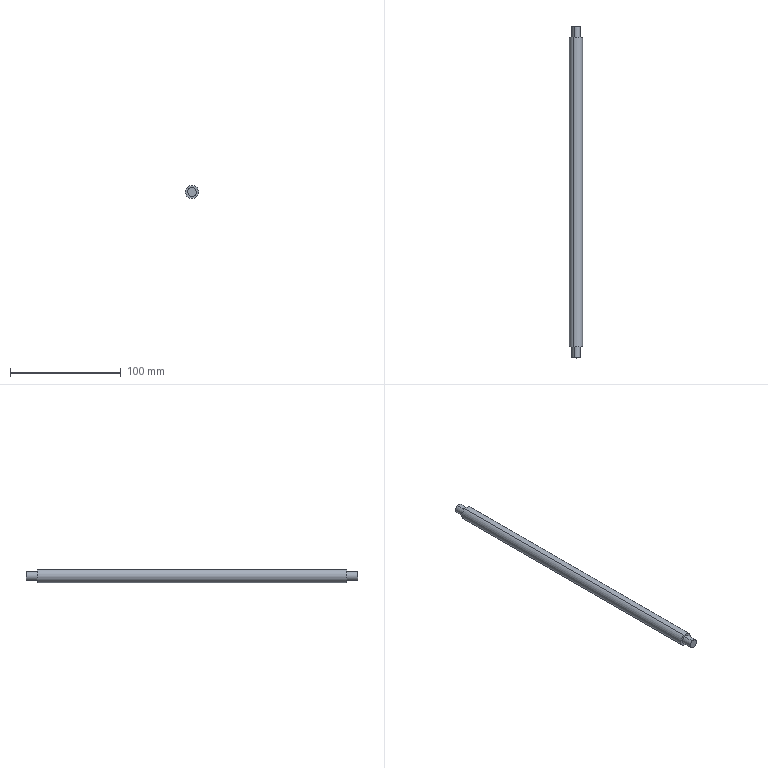Component | SolidWorks | FloatingRod-1 | 1 solid | 10 faces | box 12 x 300 x 12 mm | volume 32673 mm3 | cylinder 6 | plane 4 | commonest cylinder face diameters 8 x4 12 x2
build123d program:
from build123d import *


with BuildPart() as part:
    # Sketch1 → Revolve1 (revolve)
    with BuildSketch(Plane.XY, mode=Mode.PRIVATE) as revolve1_sk:
        Polygon((0, 150), (4, 150), (4, 140), (6, 140), (6, -140), (4, -140), (4, -150), (0, -150), align=None)
    revolve(revolve1_sk.sketch.rotate(Axis((0, 0, 0), (0, 1, 0)), 90), axis=Axis((0, 0, 0), (0, 1, 0)))


solid = part.part

# Placed as in the assembly
solid = solid.moved(Location((-15, 0, -180), (0, 0, 0)))
STEP:
#1=COLOUR_RGB('',0.7922,0.8196,0.9333);
#2=FILL_AREA_STYLE_COLOUR('',#1);
#3=FILL_AREA_STYLE('',(#2));
#4=SURFACE_STYLE_FILL_AREA(#3);
#5=SURFACE_SIDE_STYLE('',(#4));
#6=SURFACE_STYLE_USAGE(.BOTH.,#5);
#7=PRESENTATION_STYLE_ASSIGNMENT((#6));
#8=CARTESIAN_POINT('',(-0.5379,5.906,-7.235));
#9=VERTEX_POINT('',#8);
#10=CARTESIAN_POINT('',(-0.6432,5.906,-6.938));
#11=VERTEX_POINT('',#10);
#12=CARTESIAN_POINT('',(-0.5906,5.906,-7.087));
#13=DIRECTION('',(0.,-1.,-0.));
#14=DIRECTION('',(0.3341,0.,-0.9425));
#15=AXIS2_PLACEMENT_3D('',#12,#13,#14);
#16=CIRCLE('',#15,0.1575);
#17=EDGE_CURVE('',#9,#11,#16,.T.);
#18=ORIENTED_EDGE('',*,*,#17,.T.);
#19=CARTESIAN_POINT('',(-0.6432,5.512,-6.938));
#20=VERTEX_POINT('',#19);
#21=CARTESIAN_POINT('',(-0.6432,-0.,-6.938));
#22=DIRECTION('',(0.,-1.,-0.));
#23=VECTOR('',#22,39.37);
#24=LINE('',#21,#23);
#25=EDGE_CURVE('',#11,#20,#24,.T.);
#26=ORIENTED_EDGE('',*,*,#25,.T.);
#27=CARTESIAN_POINT('',(-0.5379,5.512,-7.235));
#28=VERTEX_POINT('',#27);
#29=CARTESIAN_POINT('',(-0.5906,5.512,-7.087));
#30=DIRECTION('',(0.,-1.,-0.));
#31=DIRECTION('',(0.3341,0.,-0.9425));
#32=AXIS2_PLACEMENT_3D('',#29,#30,#31);
#33=CIRCLE('',#32,0.1575);
#34=EDGE_CURVE('',#28,#20,#33,.T.);
#35=ORIENTED_EDGE('',*,*,#34,.F.);
#36=CARTESIAN_POINT('',(-0.5379,-0.,-7.235));
#37=DIRECTION('',(0.,-1.,-0.));
#38=VECTOR('',#37,39.37);
#39=LINE('',#36,#38);
#40=EDGE_CURVE('',#9,#28,#39,.T.);
#41=ORIENTED_EDGE('',*,*,#40,.F.);
#42=EDGE_LOOP('',(#18,#26,#35,#41));
#43=FACE_OUTER_BOUND('',#42,.T.);
#44=CARTESIAN_POINT('',(-0.5906,-0.,-7.087));
#45=DIRECTION('',(0.,-1.,-0.));
#46=DIRECTION('',(0.3341,0.,-0.9425));
#47=AXIS2_PLACEMENT_3D('',#44,#45,#46);
#48=CYLINDRICAL_SURFACE('',#47,0.1575);
#49=ADVANCED_FACE('',(#43),#48,.T.);
#50=CARTESIAN_POINT('',(-0.5116,5.512,-7.309));
#51=VERTEX_POINT('',#50);
#52=CARTESIAN_POINT('',(-0.6695,5.512,-6.864));
#53=VERTEX_POINT('',#52);
#54=CARTESIAN_POINT('',(-0.5906,5.512,-7.087));
#55=DIRECTION('',(0.,-1.,-0.));
#56=DIRECTION('',(0.3341,0.,-0.9425));
#57=AXIS2_PLACEMENT_3D('',#54,#55,#56);
#58=CIRCLE('',#57,0.2362);
#59=EDGE_CURVE('',#51,#53,#58,.T.);
#60=ORIENTED_EDGE('',*,*,#59,.T.);
#61=CARTESIAN_POINT('',(-0.6695,-5.512,-6.864));
#62=VERTEX_POINT('',#61);
#63=CARTESIAN_POINT('',(-0.6695,-0.,-6.864));
#64=DIRECTION('',(0.,-1.,-0.));
#65=VECTOR('',#64,39.37);
#66=LINE('',#63,#65);
#67=EDGE_CURVE('',#53,#62,#66,.T.);
#68=ORIENTED_EDGE('',*,*,#67,.T.);
#69=CARTESIAN_POINT('',(-0.5116,-5.512,-7.309));
#70=VERTEX_POINT('',#69);
#71=CARTESIAN_POINT('',(-0.5906,-5.512,-7.087));
#72=DIRECTION('',(0.,-1.,-0.));
#73=DIRECTION('',(0.3341,0.,-0.9425));
#74=AXIS2_PLACEMENT_3D('',#71,#72,#73);
#75=CIRCLE('',#74,0.2362);
#76=EDGE_CURVE('',#70,#62,#75,.T.);
#77=ORIENTED_EDGE('',*,*,#76,.F.);
#78=CARTESIAN_POINT('',(-0.5116,-0.,-7.309));
#79=DIRECTION('',(0.,-1.,-0.));
#80=VECTOR('',#79,39.37);
#81=LINE('',#78,#80);
#82=EDGE_CURVE('',#51,#70,#81,.T.);
#83=ORIENTED_EDGE('',*,*,#82,.F.);
#84=EDGE_LOOP('',(#60,#68,#77,#83));
#85=FACE_OUTER_BOUND('',#84,.T.);
#86=CARTESIAN_POINT('',(-0.5906,-0.,-7.087));
#87=DIRECTION('',(0.,-1.,-0.));
#88=DIRECTION('',(0.3341,0.,-0.9425));
#89=AXIS2_PLACEMENT_3D('',#86,#87,#88);
#90=CYLINDRICAL_SURFACE('',#89,0.2362);
#91=ADVANCED_FACE('',(#85),#90,.T.);
#92=CARTESIAN_POINT('',(-0.5379,-5.512,-7.235));
#93=VERTEX_POINT('',#92);
#94=CARTESIAN_POINT('',(-0.6432,-5.512,-6.938));
#95=VERTEX_POINT('',#94);
#96=CARTESIAN_POINT('',(-0.5906,-5.512,-7.087));
#97=DIRECTION('',(0.,-1.,-0.));
#98=DIRECTION('',(0.3341,0.,-0.9425));
#99=AXIS2_PLACEMENT_3D('',#96,#97,#98);
#100=CIRCLE('',#99,0.1575);
#101=EDGE_CURVE('',#93,#95,#100,.T.);
#102=ORIENTED_EDGE('',*,*,#101,.T.);
#103=CARTESIAN_POINT('',(-0.6432,-5.906,-6.938));
#104=VERTEX_POINT('',#103);
#105=CARTESIAN_POINT('',(-0.6432,-0.,-6.938));
#106=DIRECTION('',(0.,-1.,-0.));
#107=VECTOR('',#106,39.37);
#108=LINE('',#105,#107);
#109=EDGE_CURVE('',#95,#104,#108,.T.);
#110=ORIENTED_EDGE('',*,*,#109,.T.);
#111=CARTESIAN_POINT('',(-0.5379,-5.906,-7.235));
#112=VERTEX_POINT('',#111);
#113=CARTESIAN_POINT('',(-0.5906,-5.906,-7.087));
#114=DIRECTION('',(0.,-1.,-0.));
#115=DIRECTION('',(0.3341,0.,-0.9425));
#116=AXIS2_PLACEMENT_3D('',#113,#114,#115);
#117=CIRCLE('',#116,0.1575);
#118=EDGE_CURVE('',#112,#104,#117,.T.);
#119=ORIENTED_EDGE('',*,*,#118,.F.);
#120=CARTESIAN_POINT('',(-0.5379,-0.,-7.235));
#121=DIRECTION('',(0.,-1.,-0.));
#122=VECTOR('',#121,39.37);
#123=LINE('',#120,#122);
#124=EDGE_CURVE('',#93,#112,#123,.T.);
#125=ORIENTED_EDGE('',*,*,#124,.F.);
#126=EDGE_LOOP('',(#102,#110,#119,#125));
#127=FACE_OUTER_BOUND('',#126,.T.);
#128=CARTESIAN_POINT('',(-0.5906,-0.,-7.087));
#129=DIRECTION('',(0.,-1.,-0.));
#130=DIRECTION('',(0.3341,0.,-0.9425));
#131=AXIS2_PLACEMENT_3D('',#128,#129,#130);
#132=CYLINDRICAL_SURFACE('',#131,0.1575);
#133=ADVANCED_FACE('',(#127),#132,.T.);
#134=ORIENTED_EDGE('',*,*,#118,.T.);
#135=CARTESIAN_POINT('',(-0.5906,-5.906,-7.087));
#136=DIRECTION('',(0.,-1.,-0.));
#137=DIRECTION('',(0.3341,0.,-0.9425));
#138=AXIS2_PLACEMENT_3D('',#135,#136,#137);
#139=CIRCLE('',#138,0.1575);
#140=EDGE_CURVE('',#104,#112,#139,.T.);
#141=ORIENTED_EDGE('',*,*,#140,.T.);
#142=EDGE_LOOP('',(#134,#141));
#143=FACE_OUTER_BOUND('',#142,.T.);
#144=CARTESIAN_POINT('',(-0.5906,-5.906,-7.087));
#145=DIRECTION('',(0.,-1.,-0.));
#146=DIRECTION('',(0.3341,0.,-0.9425));
#147=AXIS2_PLACEMENT_3D('',#144,#145,#146);
#148=PLANE('',#147);
#149=ADVANCED_FACE('',(#143),#148,.T.);
#150=ORIENTED_EDGE('',*,*,#109,.F.);
#151=CARTESIAN_POINT('',(-0.5906,-5.512,-7.087));
#152=DIRECTION('',(0.,-1.,-0.));
#153=DIRECTION('',(0.3341,0.,-0.9425));
#154=AXIS2_PLACEMENT_3D('',#151,#152,#153);
#155=CIRCLE('',#154,0.1575);
#156=EDGE_CURVE('',#95,#93,#155,.T.);
#157=ORIENTED_EDGE('',*,*,#156,.T.);
#158=ORIENTED_EDGE('',*,*,#124,.T.);
#159=ORIENTED_EDGE('',*,*,#140,.F.);
#160=EDGE_LOOP('',(#150,#157,#158,#159));
#161=FACE_OUTER_BOUND('',#160,.T.);
#162=CARTESIAN_POINT('',(-0.5906,-0.,-7.087));
#163=DIRECTION('',(0.,-1.,-0.));
#164=DIRECTION('',(0.3341,0.,-0.9425));
#165=AXIS2_PLACEMENT_3D('',#162,#163,#164);
#166=CYLINDRICAL_SURFACE('',#165,0.1575);
#167=ADVANCED_FACE('',(#161),#166,.T.);
#168=ORIENTED_EDGE('',*,*,#76,.T.);
#169=CARTESIAN_POINT('',(-0.5906,-5.512,-7.087));
#170=DIRECTION('',(0.,-1.,-0.));
#171=DIRECTION('',(0.3341,0.,-0.9425));
#172=AXIS2_PLACEMENT_3D('',#169,#170,#171);
#173=CIRCLE('',#172,0.2362);
#174=EDGE_CURVE('',#62,#70,#173,.T.);
#175=ORIENTED_EDGE('',*,*,#174,.T.);
#176=EDGE_LOOP('',(#168,#175));
#177=FACE_OUTER_BOUND('',#176,.T.);
#178=ORIENTED_EDGE('',*,*,#101,.F.);
#179=ORIENTED_EDGE('',*,*,#156,.F.);
#180=EDGE_LOOP('',(#178,#179));
#181=FACE_BOUND('',#180,.T.);
#182=CARTESIAN_POINT('',(-0.4421,-5.512,-7.034));
#183=DIRECTION('',(0.,-1.,-0.));
#184=DIRECTION('',(0.3341,0.,-0.9425));
#185=AXIS2_PLACEMENT_3D('',#182,#183,#184);
#186=PLANE('',#185);
#187=ADVANCED_FACE('',(#177,#181),#186,.T.);
#188=ORIENTED_EDGE('',*,*,#67,.F.);
#189=CARTESIAN_POINT('',(-0.5906,5.512,-7.087));
#190=DIRECTION('',(0.,-1.,-0.));
#191=DIRECTION('',(0.3341,0.,-0.9425));
#192=AXIS2_PLACEMENT_3D('',#189,#190,#191);
#193=CIRCLE('',#192,0.2362);
#194=EDGE_CURVE('',#53,#51,#193,.T.);
#195=ORIENTED_EDGE('',*,*,#194,.T.);
#196=ORIENTED_EDGE('',*,*,#82,.T.);
#197=ORIENTED_EDGE('',*,*,#174,.F.);
#198=EDGE_LOOP('',(#188,#195,#196,#197));
#199=FACE_OUTER_BOUND('',#198,.T.);
#200=CARTESIAN_POINT('',(-0.5906,-0.,-7.087));
#201=DIRECTION('',(0.,-1.,-0.));
#202=DIRECTION('',(0.3341,0.,-0.9425));
#203=AXIS2_PLACEMENT_3D('',#200,#201,#202);
#204=CYLINDRICAL_SURFACE('',#203,0.2362);
#205=ADVANCED_FACE('',(#199),#204,.T.);
#206=ORIENTED_EDGE('',*,*,#34,.T.);
#207=CARTESIAN_POINT('',(-0.5906,5.512,-7.087));
#208=DIRECTION('',(0.,-1.,-0.));
#209=DIRECTION('',(0.3341,0.,-0.9425));
#210=AXIS2_PLACEMENT_3D('',#207,#208,#209);
#211=CIRCLE('',#210,0.1575);
#212=EDGE_CURVE('',#20,#28,#211,.T.);
#213=ORIENTED_EDGE('',*,*,#212,.T.);
#214=EDGE_LOOP('',(#206,#213));
#215=FACE_BOUND('',#214,.T.);
#216=ORIENTED_EDGE('',*,*,#59,.F.);
#217=ORIENTED_EDGE('',*,*,#194,.F.);
#218=EDGE_LOOP('',(#216,#217));
#219=FACE_OUTER_BOUND('',#218,.T.);
#220=CARTESIAN_POINT('',(-0.4421,5.512,-7.034));
#221=DIRECTION('',(-0.,1.,0.));
#222=DIRECTION('',(-0.3341,-0.,0.9425));
#223=AXIS2_PLACEMENT_3D('',#220,#221,#222);
#224=PLANE('',#223);
#225=ADVANCED_FACE('',(#215,#219),#224,.T.);
#226=ORIENTED_EDGE('',*,*,#25,.F.);
#227=CARTESIAN_POINT('',(-0.5906,5.906,-7.087));
#228=DIRECTION('',(0.,-1.,-0.));
#229=DIRECTION('',(0.3341,0.,-0.9425));
#230=AXIS2_PLACEMENT_3D('',#227,#228,#229);
#231=CIRCLE('',#230,0.1575);
#232=EDGE_CURVE('',#11,#9,#231,.T.);
#233=ORIENTED_EDGE('',*,*,#232,.T.);
#234=ORIENTED_EDGE('',*,*,#40,.T.);
#235=ORIENTED_EDGE('',*,*,#212,.F.);
#236=EDGE_LOOP('',(#226,#233,#234,#235));
#237=FACE_OUTER_BOUND('',#236,.T.);
#238=CARTESIAN_POINT('',(-0.5906,-0.,-7.087));
#239=DIRECTION('',(0.,-1.,-0.));
#240=DIRECTION('',(0.3341,0.,-0.9425));
#241=AXIS2_PLACEMENT_3D('',#238,#239,#240);
#242=CYLINDRICAL_SURFACE('',#241,0.1575);
#243=ADVANCED_FACE('',(#237),#242,.T.);
#244=ORIENTED_EDGE('',*,*,#17,.F.);
#245=ORIENTED_EDGE('',*,*,#232,.F.);
#246=EDGE_LOOP('',(#244,#245));
#247=FACE_OUTER_BOUND('',#246,.T.);
#248=CARTESIAN_POINT('',(-0.5906,5.906,-7.087));
#249=DIRECTION('',(-0.,1.,0.));
#250=DIRECTION('',(-0.3341,-0.,0.9425));
#251=AXIS2_PLACEMENT_3D('',#248,#249,#250);
#252=PLANE('',#251);
#253=ADVANCED_FACE('',(#247),#252,.T.);
#254=CLOSED_SHELL('',(#49,#91,#133,#149,#167,#187,#205,#225,#243,#253));
#255=MANIFOLD_SOLID_BREP('',#254);
#256=STYLED_ITEM('',(#7),#255);
#257=PRESENTATION_LAYER_ASSIGNMENT('','',(#256));
#258=CARTESIAN_POINT('',(0.,0.,0.));
#259=DIRECTION('',(0.,0.,1.));
#260=DIRECTION('',(1.,0.,0.));
#261=AXIS2_PLACEMENT_3D('',#258,#259,#260);
#262=(LENGTH_UNIT()NAMED_UNIT(*)SI_UNIT($,.METRE.));
#263=LENGTH_MEASURE_WITH_UNIT(LENGTH_MEASURE(0.0254),#262);
#264=DIMENSIONAL_EXPONENTS(1.,0.,0.,0.,0.,0.,0.);
#265=(CONVERSION_BASED_UNIT('',#263)LENGTH_UNIT()NAMED_UNIT(#264));
#266=UNCERTAINTY_MEASURE_WITH_UNIT(LENGTH_MEASURE(0.00001),#265,'','');
#267=(NAMED_UNIT(*)PLANE_ANGLE_UNIT()SI_UNIT($,.RADIAN.));
#268=(NAMED_UNIT(*)SI_UNIT($,.STERADIAN.)SOLID_ANGLE_UNIT());
#269=(GEOMETRIC_REPRESENTATION_CONTEXT(3)GLOBAL_UNCERTAINTY_ASSIGNED_CONTEXT((#266))GLOBAL_UNIT_ASSIGNED_CONTEXT((#265,#267,#268))REPRESENTATION_CONTEXT('',''));
#270=ADVANCED_BREP_SHAPE_REPRESENTATION('',(#255,#261),#269);
#271=(LENGTH_UNIT()NAMED_UNIT(*)SI_UNIT($,.METRE.));
#272=LENGTH_MEASURE_WITH_UNIT(LENGTH_MEASURE(0.0254),#271);
#273=DIMENSIONAL_EXPONENTS(1.,0.,0.,0.,0.,0.,0.);
#274=(CONVERSION_BASED_UNIT('',#272)LENGTH_UNIT()NAMED_UNIT(#273));
#275=UNCERTAINTY_MEASURE_WITH_UNIT(LENGTH_MEASURE(0.00001),#274,'','');
#276=(NAMED_UNIT(*)PLANE_ANGLE_UNIT()SI_UNIT($,.RADIAN.));
#277=(NAMED_UNIT(*)SI_UNIT($,.STERADIAN.)SOLID_ANGLE_UNIT());
#278=(GEOMETRIC_REPRESENTATION_CONTEXT(3)GLOBAL_UNCERTAINTY_ASSIGNED_CONTEXT((#275))GLOBAL_UNIT_ASSIGNED_CONTEXT((#274,#276,#277))REPRESENTATION_CONTEXT('',''));
#279=MECHANICAL_DESIGN_GEOMETRIC_PRESENTATION_REPRESENTATION('',(#256),#278);